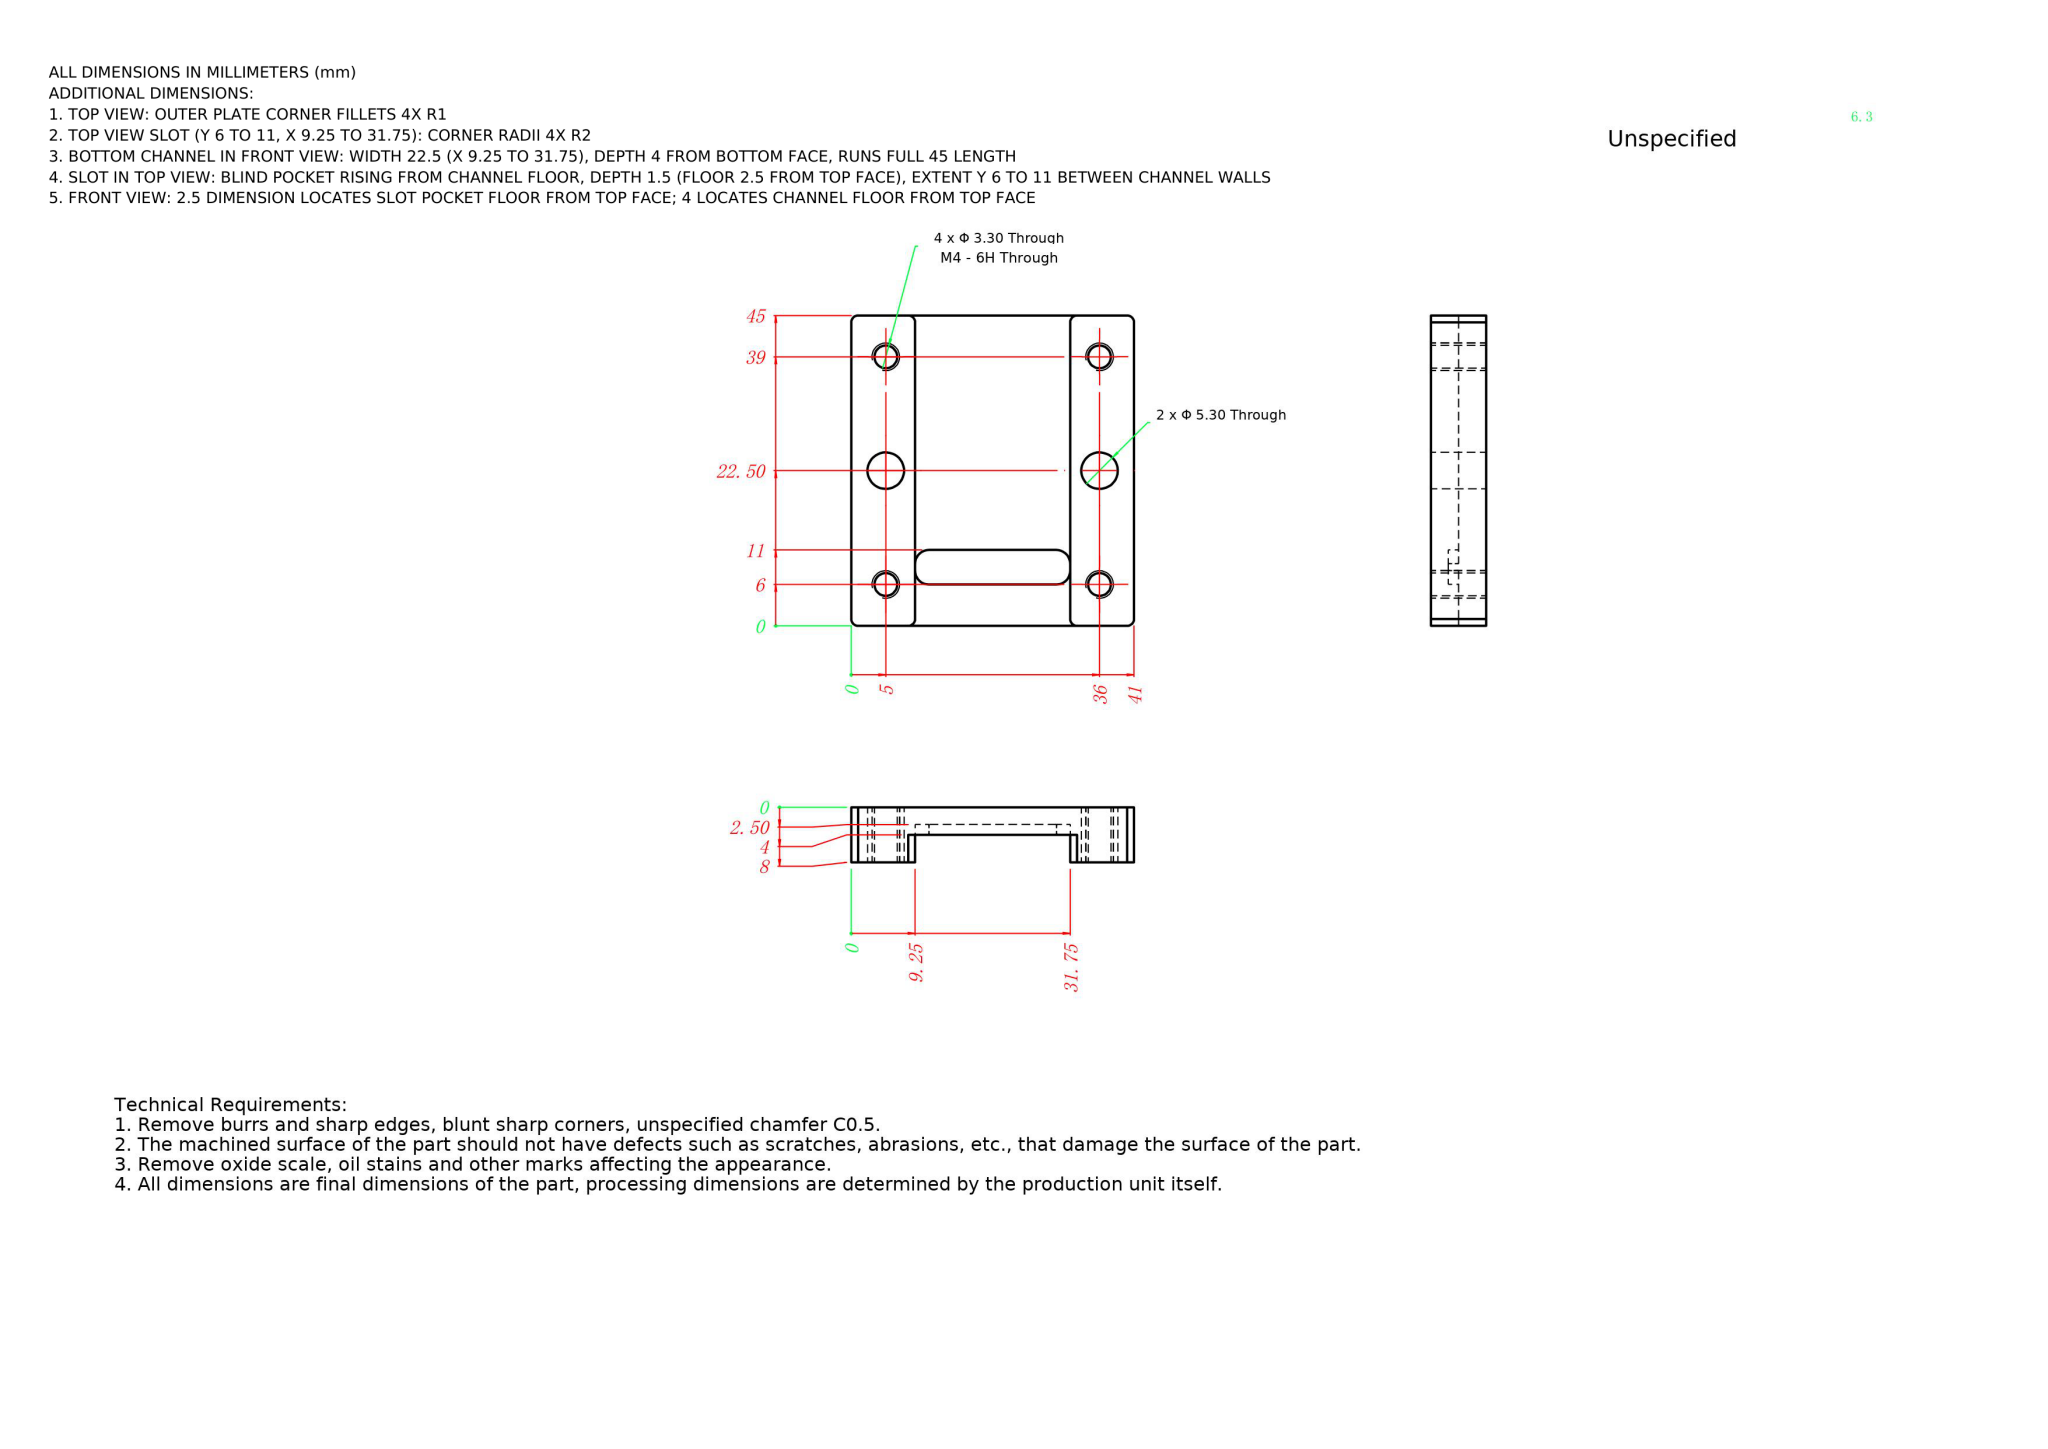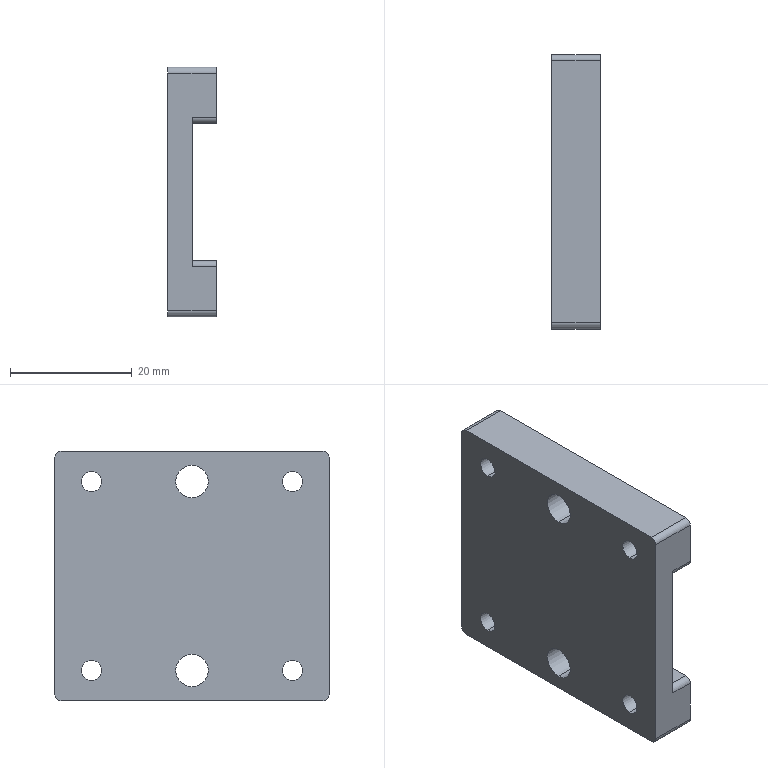Part | NX | mm | 1 solid | 38 faces | box 8 x 45 x 41 mm | volume 9909 mm3 | cylinder 24 | plane 14 | commonest cylinder face diameters 3.3 x8 2 x8 5.3 x4 4 x4